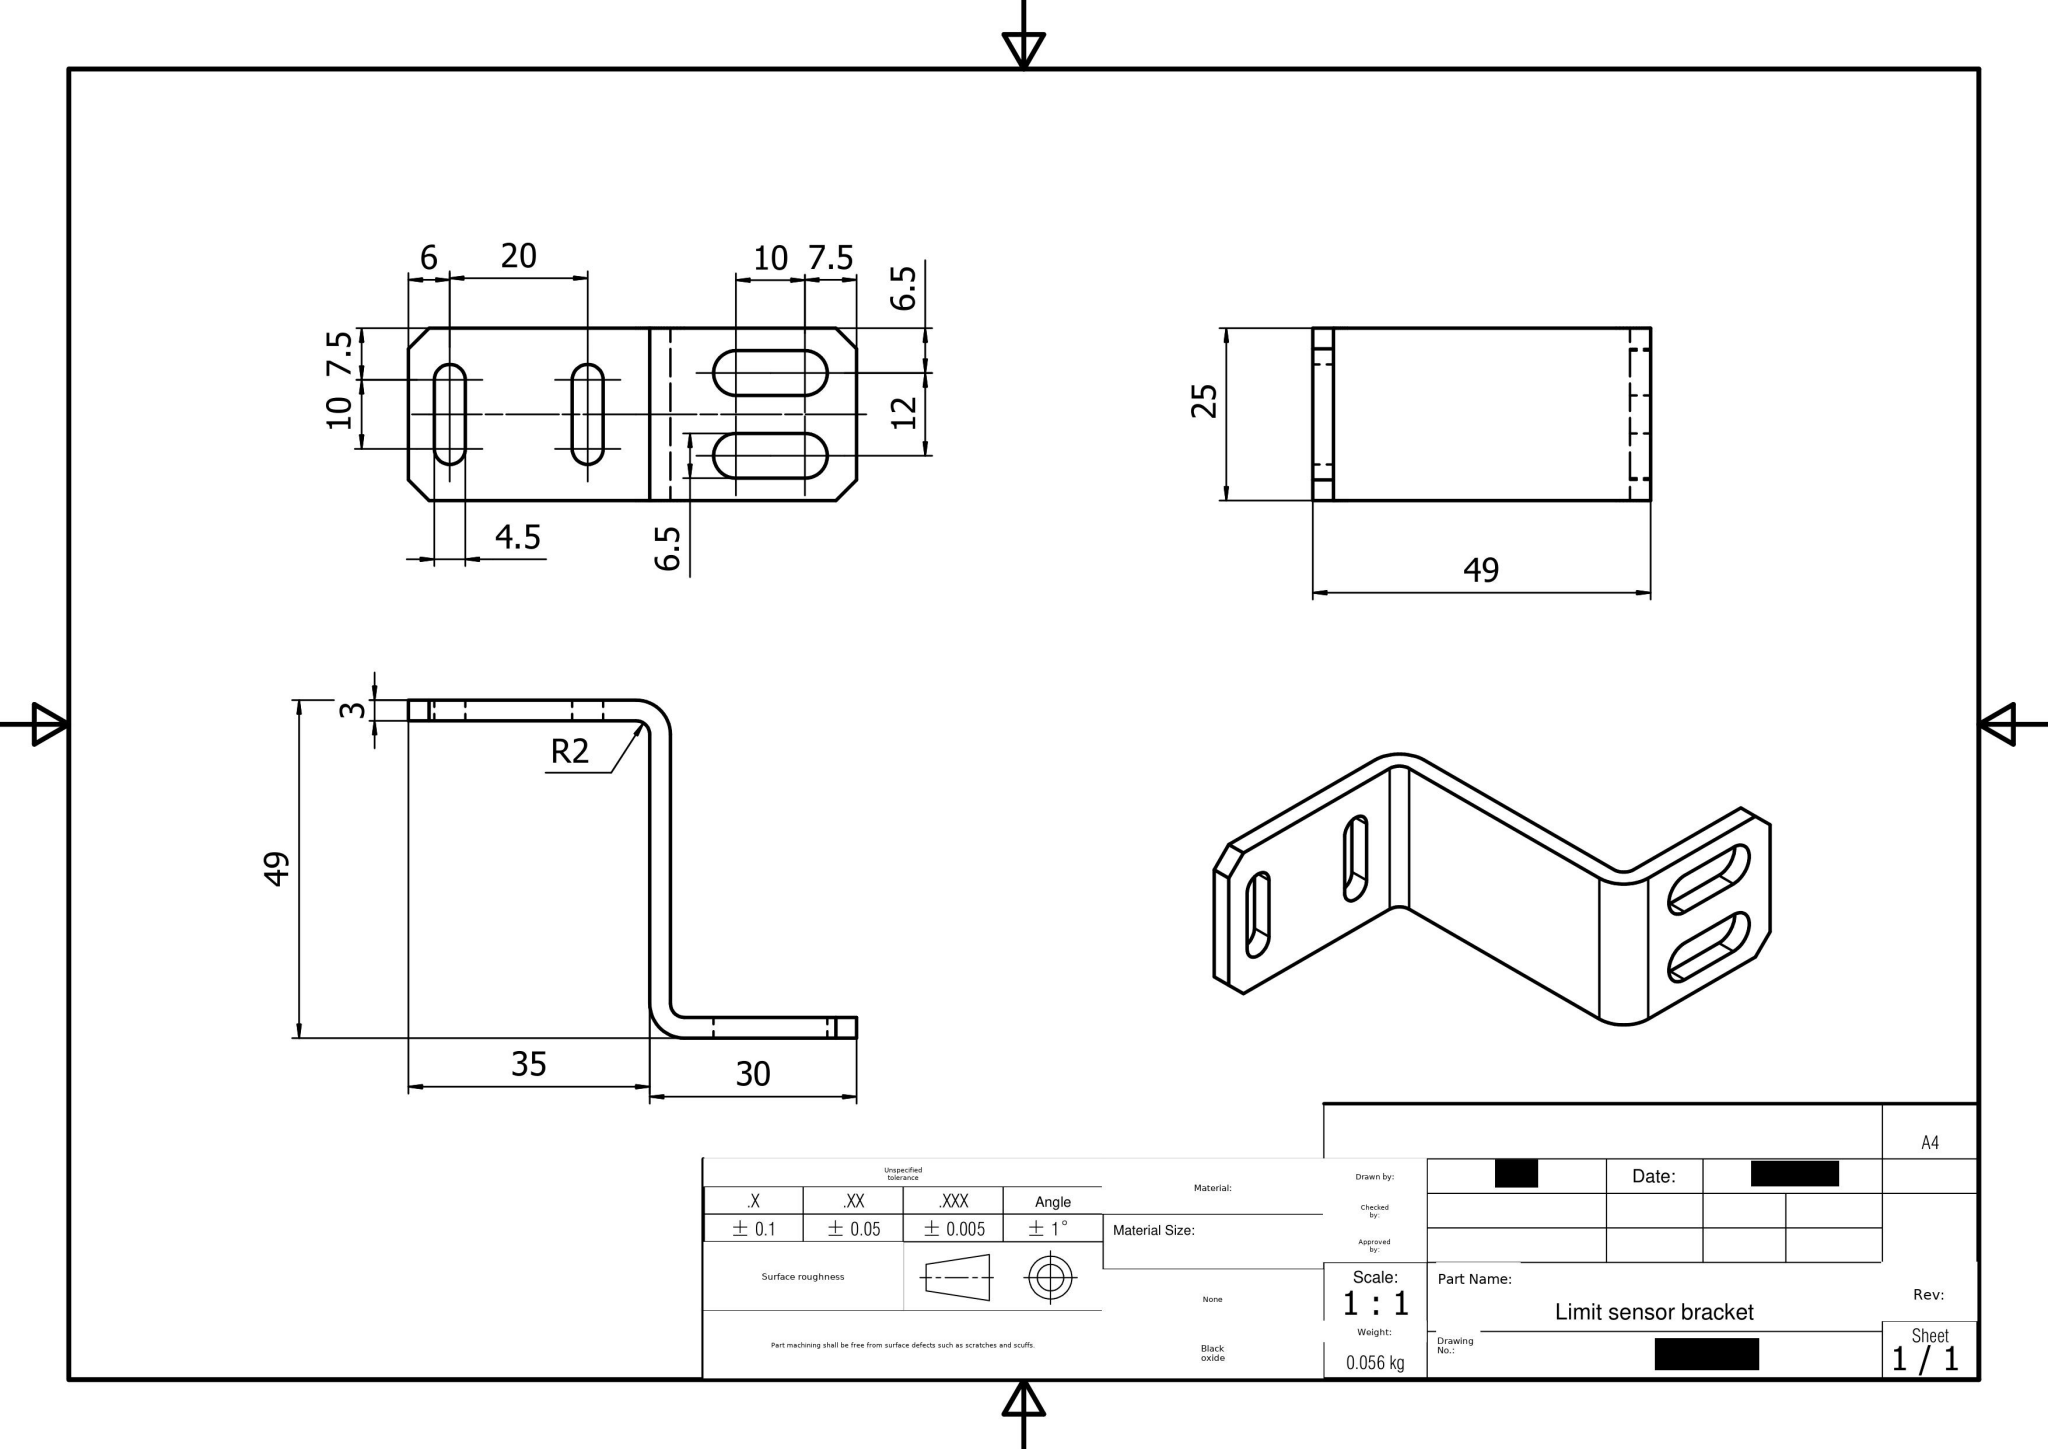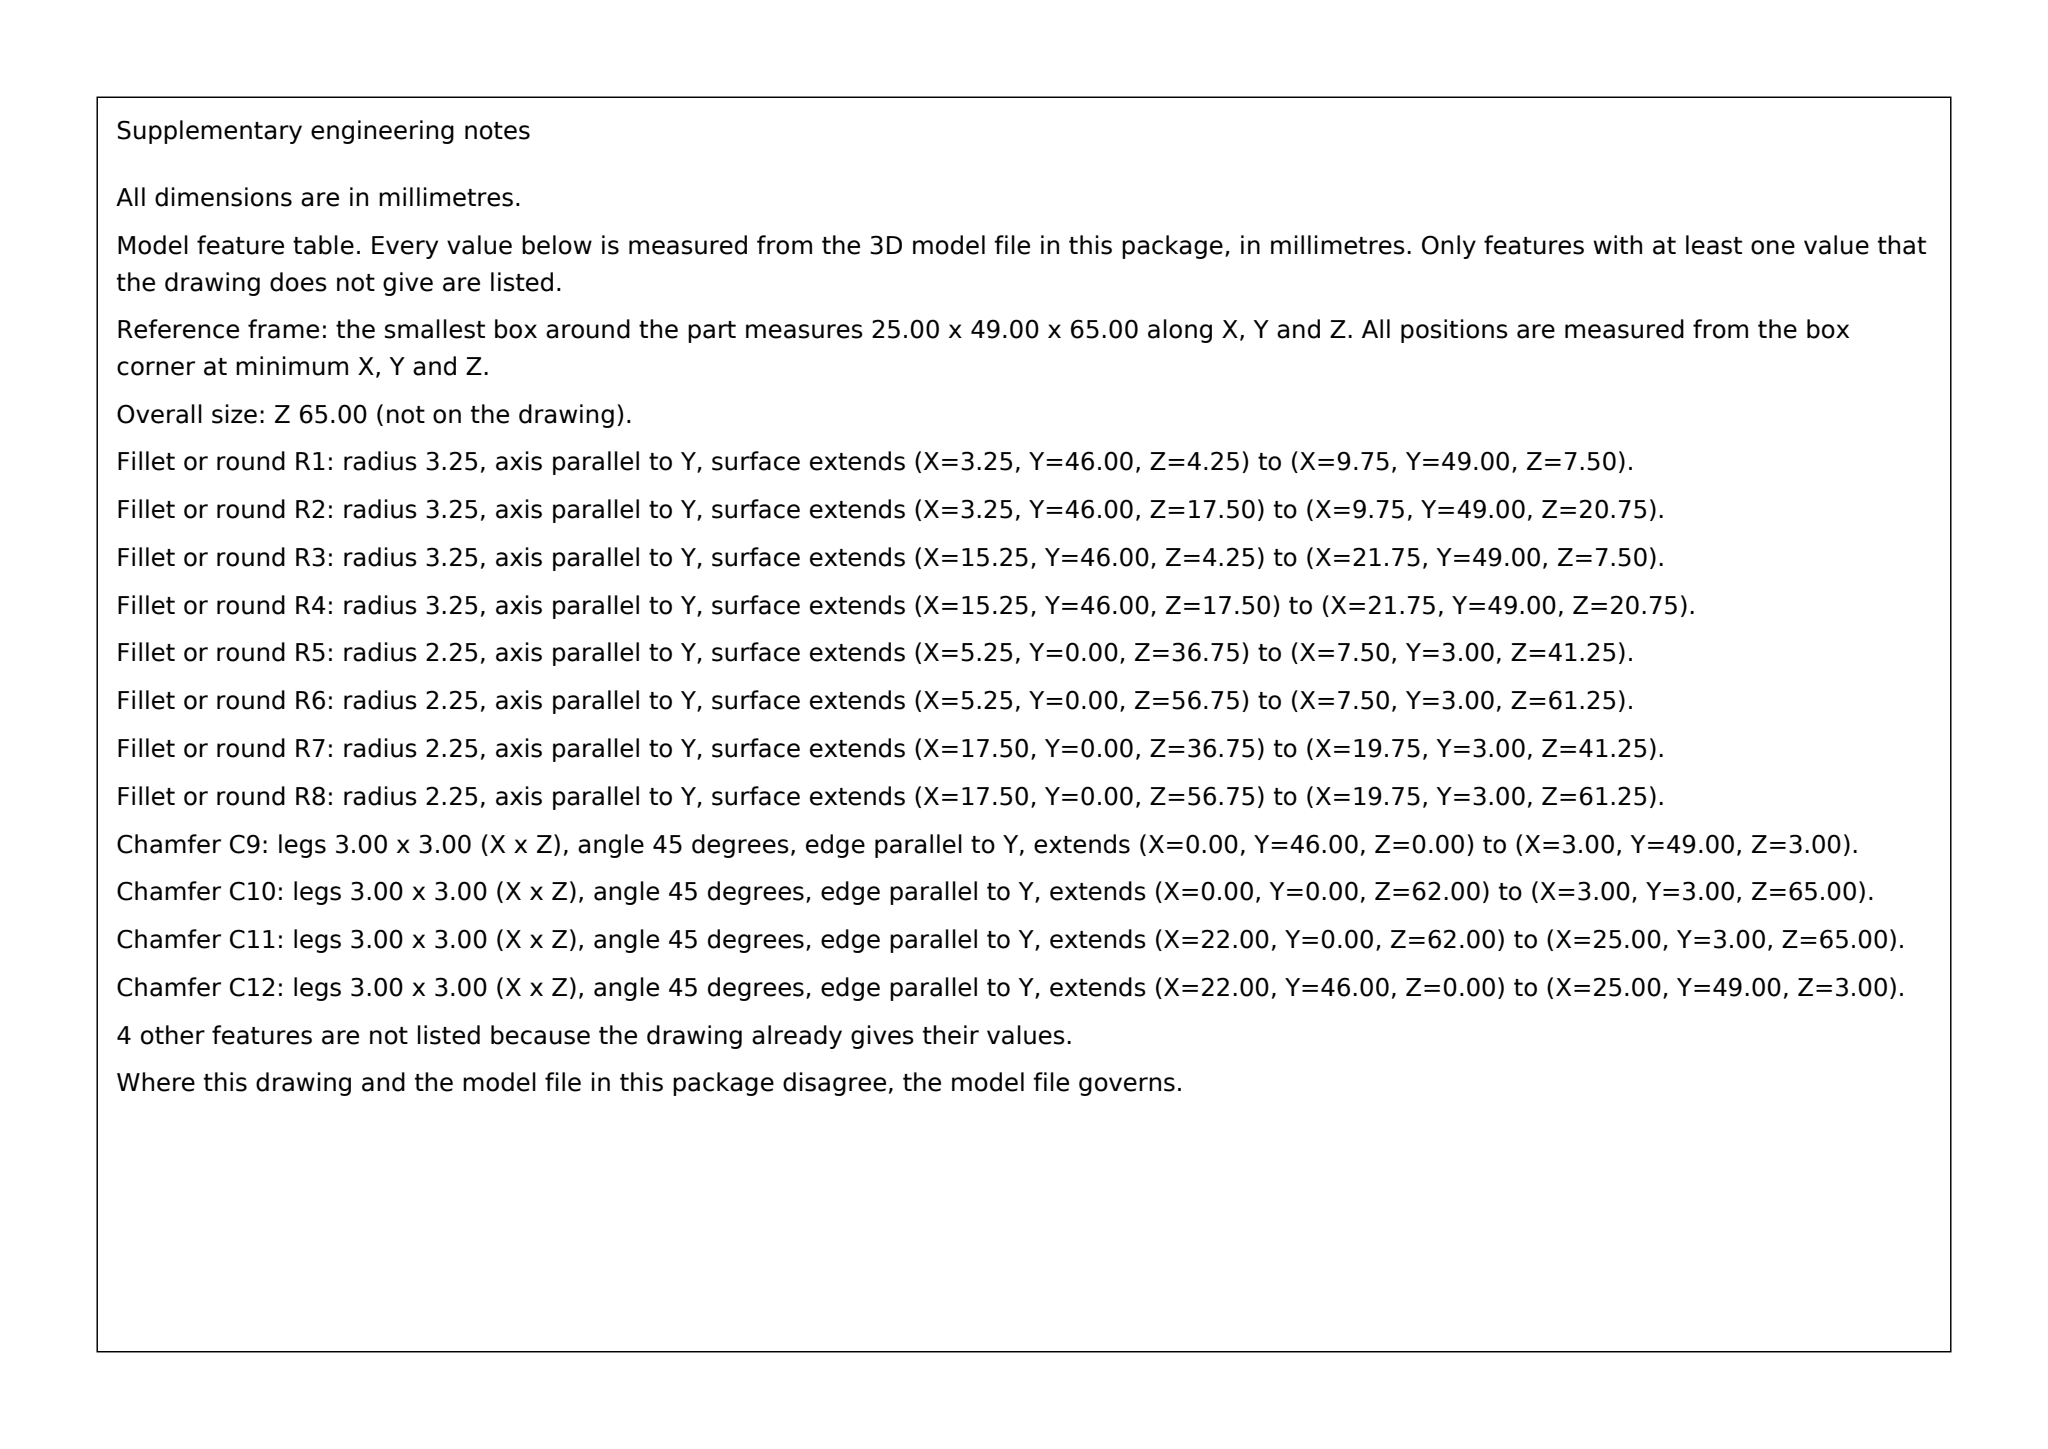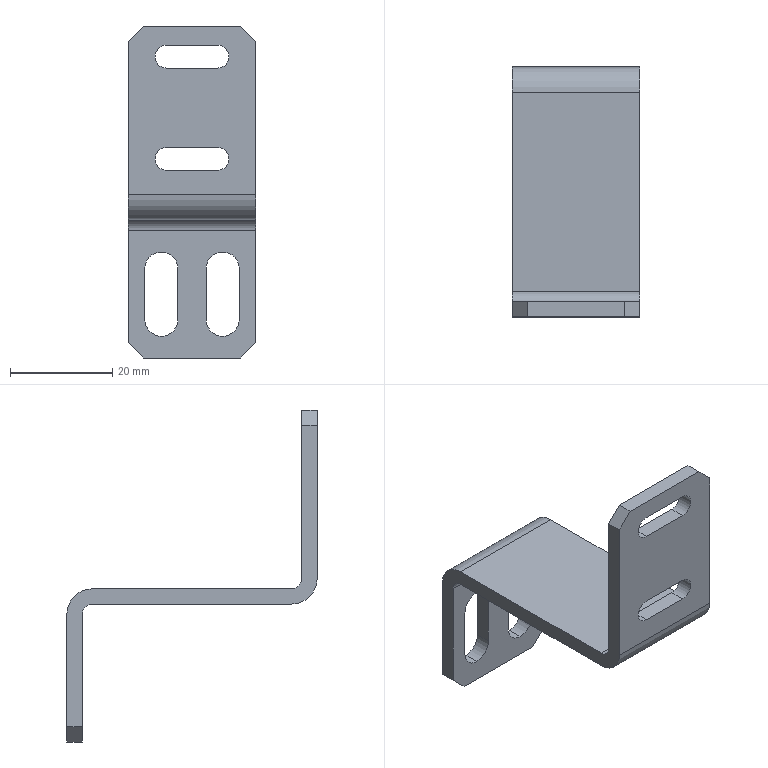Part | SolidWorks | mm | 1 solid | 36 faces | box 25 x 49 x 65 mm | volume 7091 mm3 | plane 22 | cylinder 14 | commonest cylinder face diameters 6.5 x6 4.5 x4 10 x2 4 x2